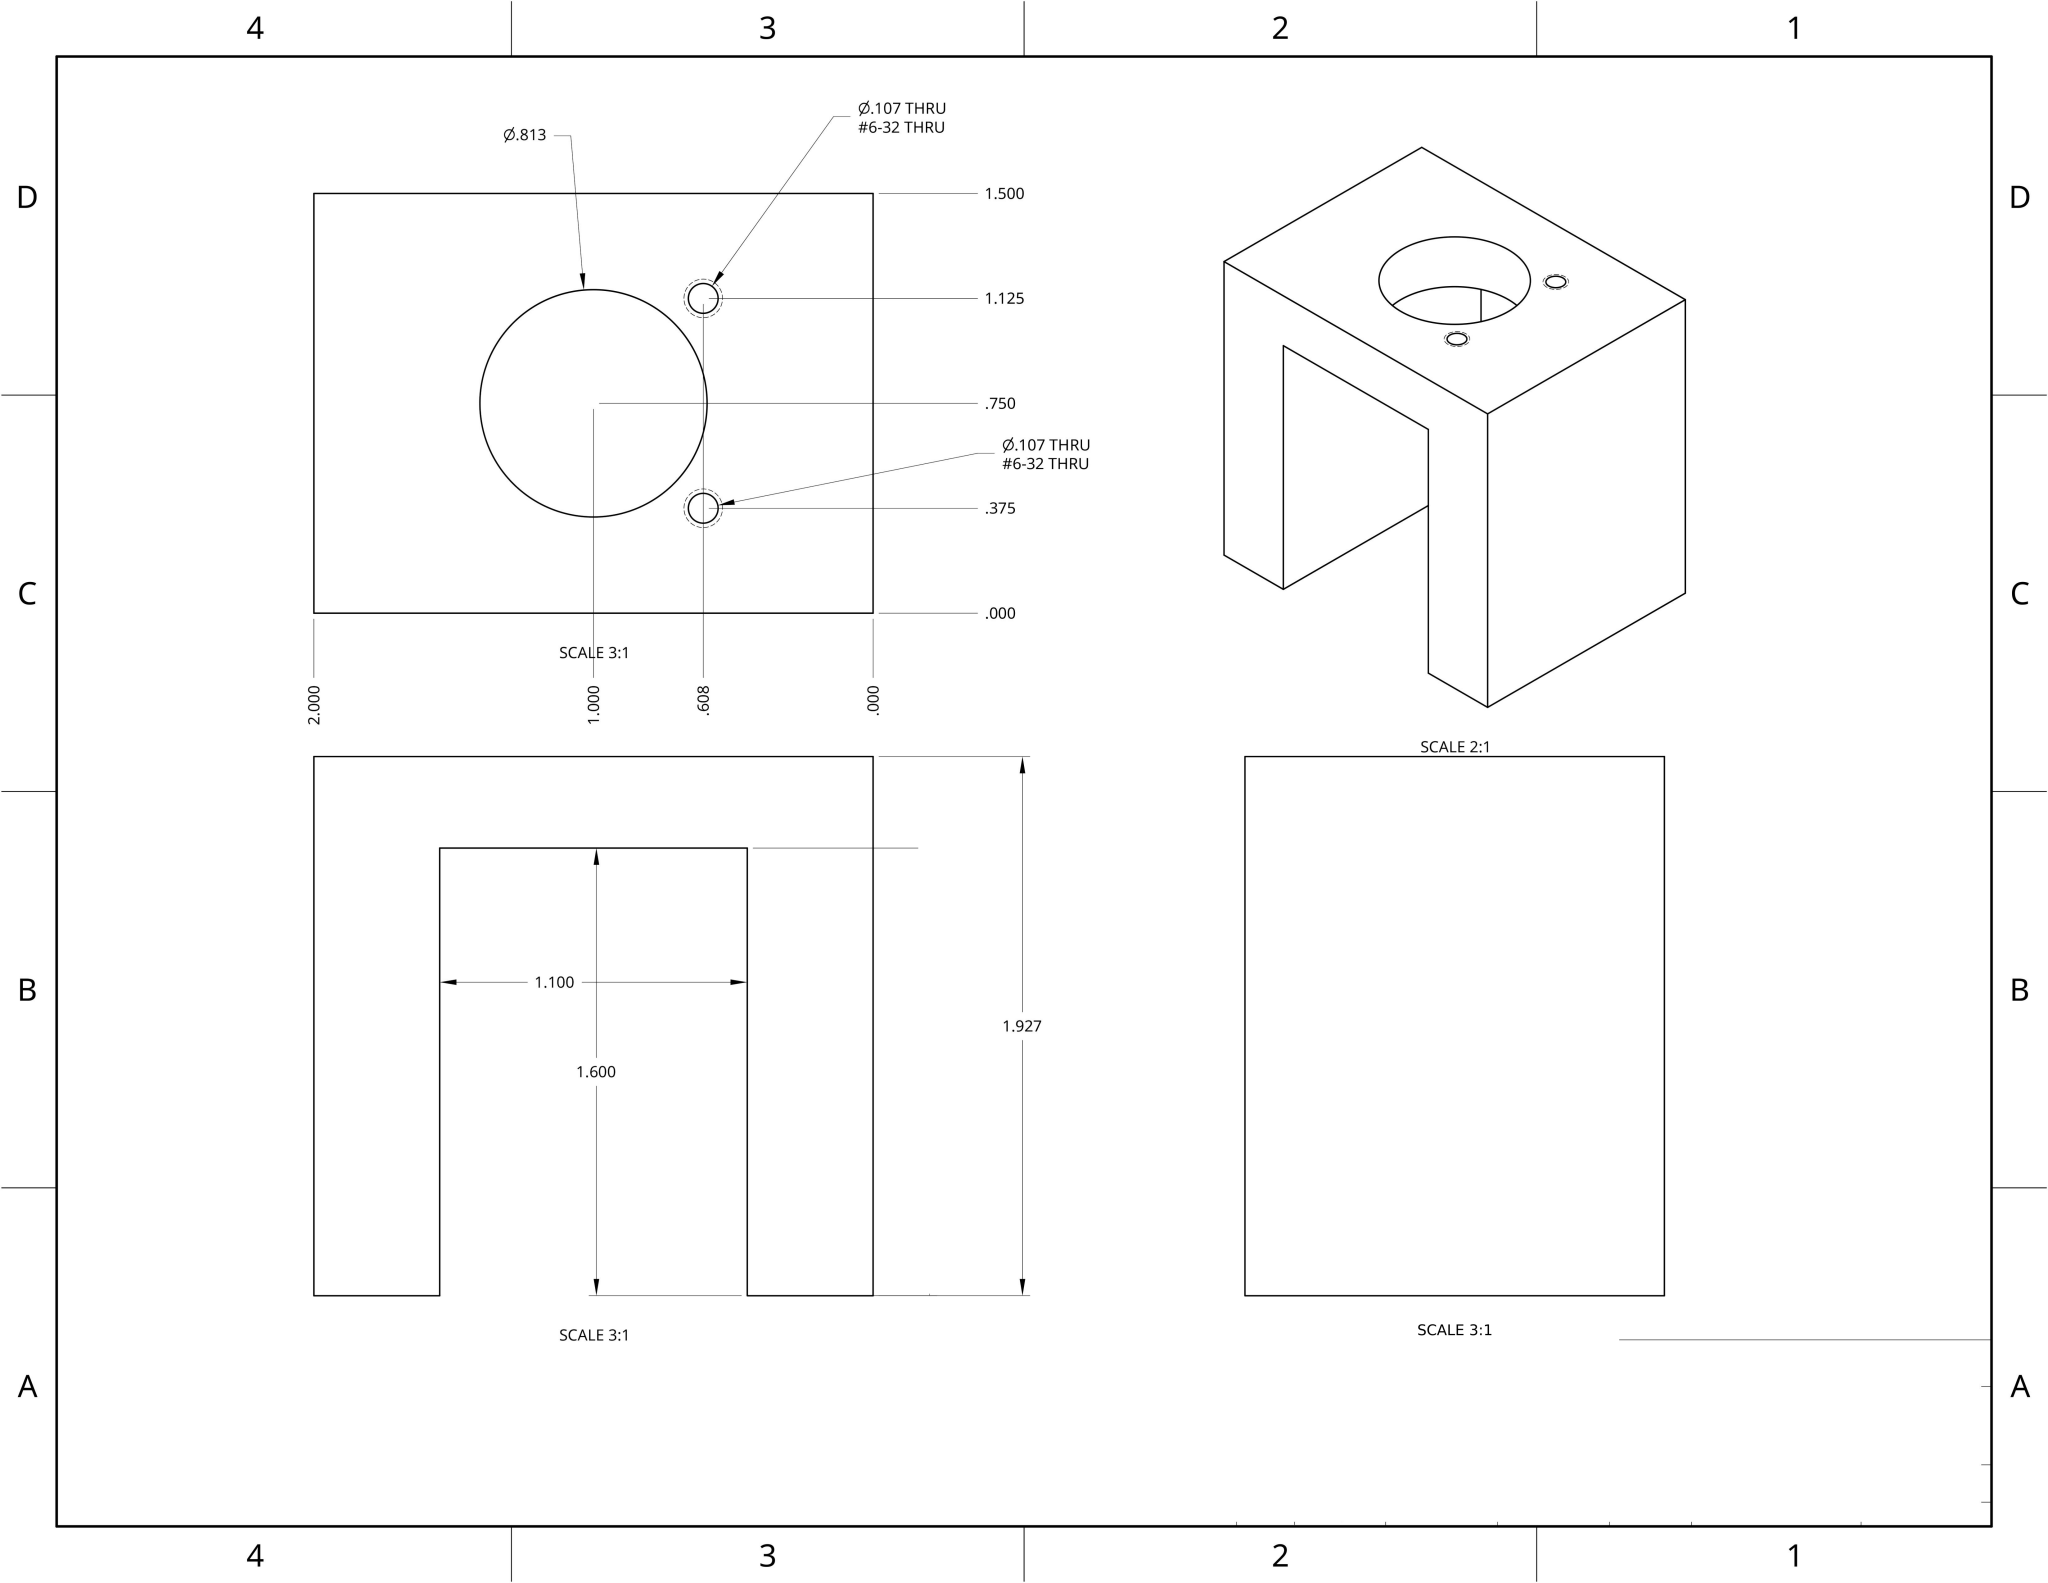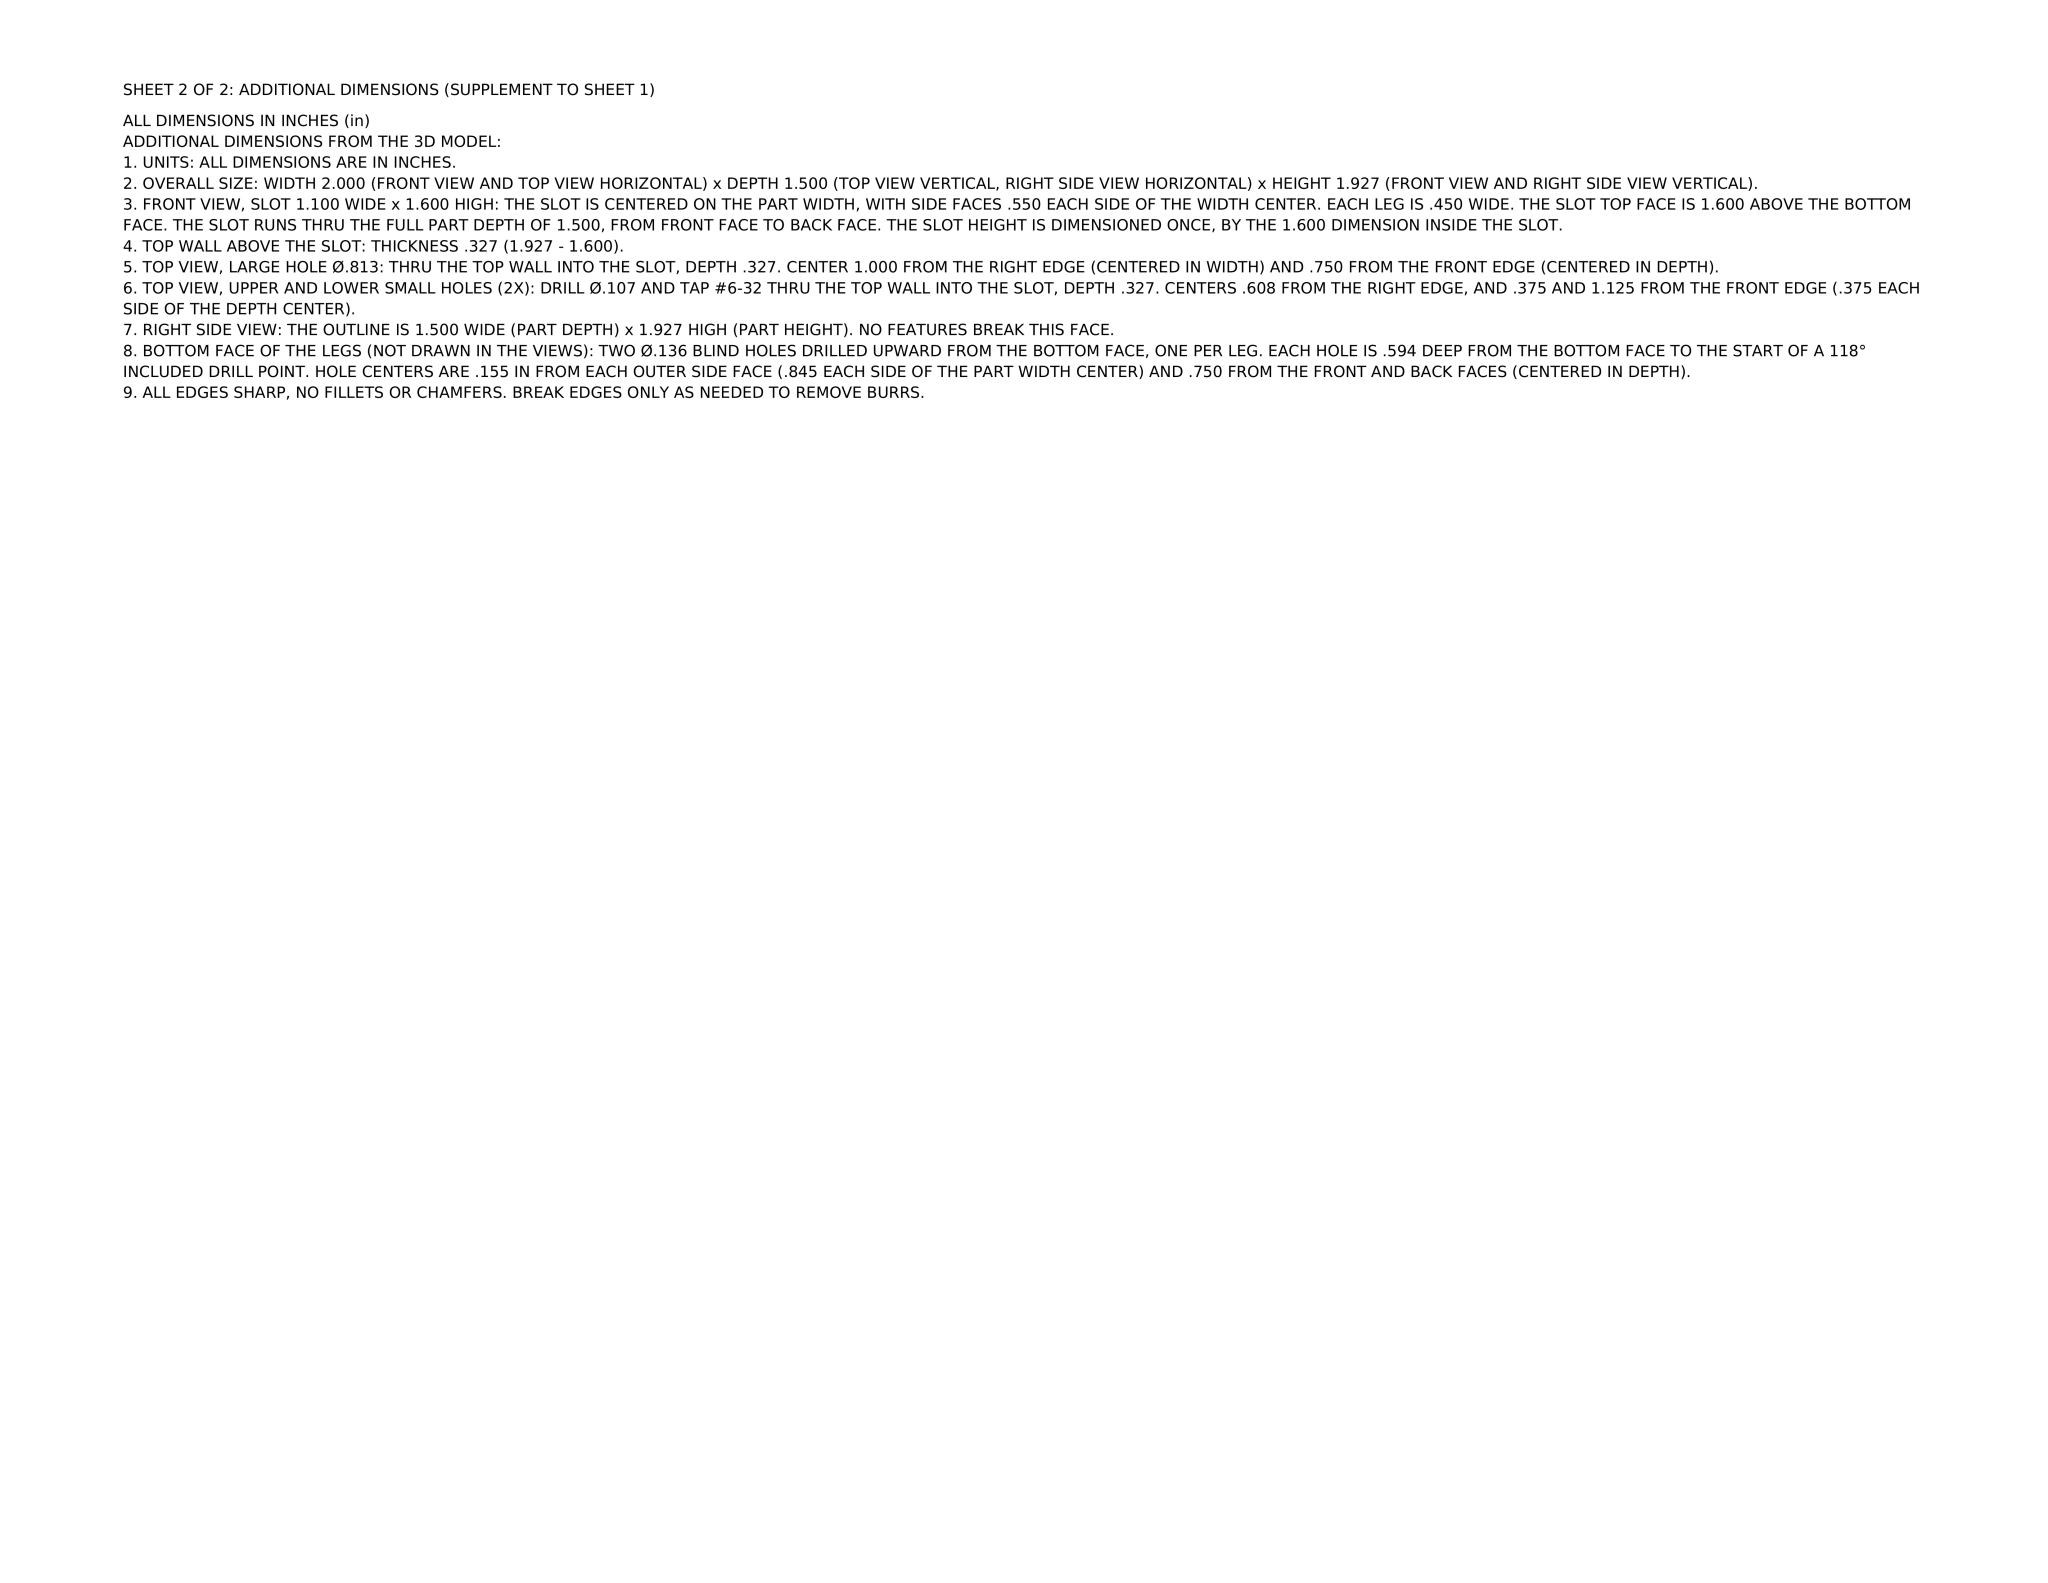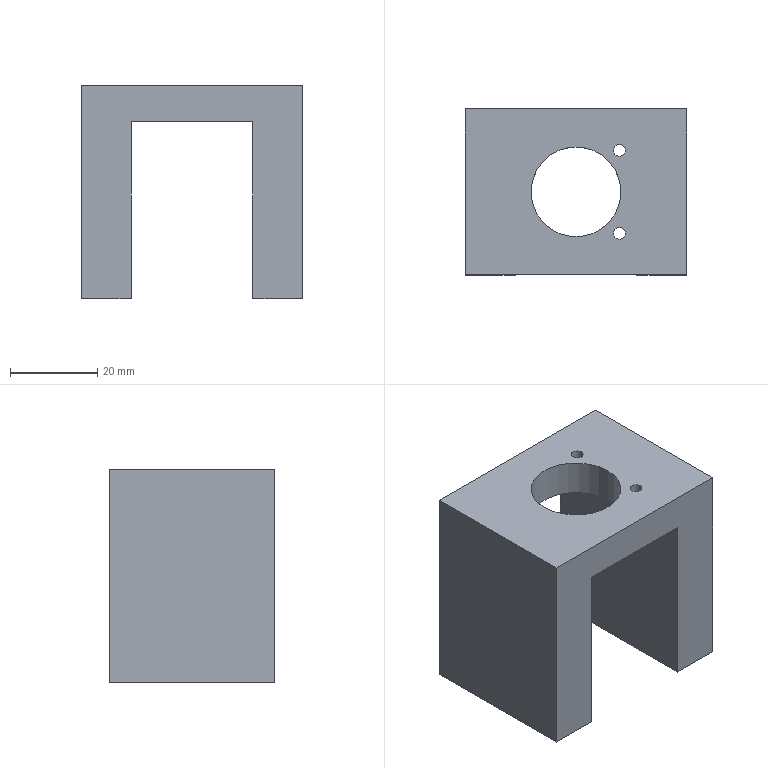Part | NX | drawing in metres | 1 solid | 17 faces | box 50.8 x 38.1 x 48.95 mm | volume 48309 mm3 | plane 10 | cylinder 5 | cone 2 | commonest cylinder face diameters 2.705 x2 3.454 x2 20.637 x1
STEP:
#1=COLOUR_RGB('',0.6039,0.6471,0.6863);
#2=FILL_AREA_STYLE_COLOUR('',#1);
#3=FILL_AREA_STYLE('',(#2));
#4=SURFACE_STYLE_FILL_AREA(#3);
#5=SURFACE_SIDE_STYLE('',(#4));
#6=SURFACE_STYLE_USAGE(.BOTH.,#5);
#7=PRESENTATION_STYLE_ASSIGNMENT((#6));
#8=CARTESIAN_POINT('',(0.01132,-0.009525,0.04895));
#9=VERTEX_POINT('',#8);
#10=CARTESIAN_POINT('',(0.009969,-0.009525,0.04895));
#11=DIRECTION('',(0.,0.,1.));
#12=DIRECTION('',(1.,0.,0.));
#13=AXIS2_PLACEMENT_3D('',#10,#11,#12);
#14=CIRCLE('',#13,0.001353);
#15=EDGE_CURVE('',#9,#9,#14,.F.);
#16=ORIENTED_EDGE('',*,*,#15,.F.);
#17=EDGE_LOOP('',(#16));
#18=FACE_OUTER_BOUND('',#17,.T.);
#19=CARTESIAN_POINT('',(0.01132,-0.009525,0.04064));
#20=VERTEX_POINT('',#19);
#21=CARTESIAN_POINT('',(0.009969,-0.009525,0.04064));
#22=DIRECTION('',(0.,0.,1.));
#23=DIRECTION('',(1.,0.,-0.));
#24=AXIS2_PLACEMENT_3D('',#21,#22,#23);
#25=CIRCLE('',#24,0.001353);
#26=EDGE_CURVE('',#20,#20,#25,.F.);
#27=ORIENTED_EDGE('',*,*,#26,.T.);
#28=EDGE_LOOP('',(#27));
#29=FACE_OUTER_BOUND('',#28,.T.);
#30=CARTESIAN_POINT('',(0.009969,-0.009525,0.08058));
#31=DIRECTION('',(0.,0.,1.));
#32=DIRECTION('',(-1.,0.,0.));
#33=AXIS2_PLACEMENT_3D('',#30,#31,#32);
#34=CYLINDRICAL_SURFACE('',#33,0.001353);
#35=ADVANCED_FACE('',(#18,#29),#34,.F.);
#36=STYLED_ITEM('',(#7),#35);
#37=COLOUR_RGB('',0.6039,0.6471,0.6863);
#38=FILL_AREA_STYLE_COLOUR('',#37);
#39=FILL_AREA_STYLE('',(#38));
#40=SURFACE_STYLE_FILL_AREA(#39);
#41=SURFACE_SIDE_STYLE('',(#40));
#42=SURFACE_STYLE_USAGE(.BOTH.,#41);
#43=PRESENTATION_STYLE_ASSIGNMENT((#42));
#44=CARTESIAN_POINT('',(-0.0254,0.01905,0.));
#45=VERTEX_POINT('',#44);
#46=CARTESIAN_POINT('',(-0.0254,-0.01905,0.));
#47=VERTEX_POINT('',#46);
#48=CARTESIAN_POINT('',(-0.0254,-0.004293,0.));
#49=DIRECTION('',(0.,-1.,0.));
#50=VECTOR('',#49,1.);
#51=LINE('',#48,#50);
#52=EDGE_CURVE('',#45,#47,#51,.T.);
#53=ORIENTED_EDGE('',*,*,#52,.T.);
#54=CARTESIAN_POINT('',(-0.0254,-0.01905,0.04895));
#55=VERTEX_POINT('',#54);
#56=CARTESIAN_POINT('',(-0.0254,-0.01905,0.04895));
#57=DIRECTION('',(0.,0.,-1.));
#58=VECTOR('',#57,1.);
#59=LINE('',#56,#58);
#60=EDGE_CURVE('',#55,#47,#59,.T.);
#61=ORIENTED_EDGE('',*,*,#60,.F.);
#62=CARTESIAN_POINT('',(-0.0254,0.01905,0.04895));
#63=VERTEX_POINT('',#62);
#64=CARTESIAN_POINT('',(-0.0254,-0.004293,0.04895));
#65=DIRECTION('',(0.,-1.,0.));
#66=VECTOR('',#65,1.);
#67=LINE('',#64,#66);
#68=EDGE_CURVE('',#63,#55,#67,.T.);
#69=ORIENTED_EDGE('',*,*,#68,.F.);
#70=CARTESIAN_POINT('',(-0.0254,0.01905,0.04895));
#71=DIRECTION('',(0.,0.,-1.));
#72=VECTOR('',#71,1.);
#73=LINE('',#70,#72);
#74=EDGE_CURVE('',#63,#45,#73,.T.);
#75=ORIENTED_EDGE('',*,*,#74,.T.);
#76=EDGE_LOOP('',(#53,#61,#69,#75));
#77=FACE_OUTER_BOUND('',#76,.T.);
#78=CARTESIAN_POINT('',(-0.0254,-0.004293,0.04895));
#79=DIRECTION('',(1.,0.,0.));
#80=DIRECTION('',(0.,0.,-1.));
#81=AXIS2_PLACEMENT_3D('',#78,#79,#80);
#82=PLANE('',#81);
#83=ADVANCED_FACE('',(#77),#82,.F.);
#84=STYLED_ITEM('',(#43),#83);
#85=COLOUR_RGB('',0.6039,0.6471,0.6863);
#86=FILL_AREA_STYLE_COLOUR('',#85);
#87=FILL_AREA_STYLE('',(#86));
#88=SURFACE_STYLE_FILL_AREA(#87);
#89=SURFACE_SIDE_STYLE('',(#88));
#90=SURFACE_STYLE_USAGE(.BOTH.,#89);
#91=PRESENTATION_STYLE_ASSIGNMENT((#90));
#92=CARTESIAN_POINT('',(0.01974,-0.,0.));
#93=VERTEX_POINT('',#92);
#94=CARTESIAN_POINT('',(0.02146,-0.,0.));
#95=DIRECTION('',(0.,0.,-1.));
#96=DIRECTION('',(-1.,0.,0.));
#97=AXIS2_PLACEMENT_3D('',#94,#95,#96);
#98=CIRCLE('',#97,0.001727);
#99=EDGE_CURVE('',#93,#93,#98,.T.);
#100=ORIENTED_EDGE('',*,*,#99,.F.);
#101=EDGE_LOOP('',(#100));
#102=FACE_BOUND('',#101,.T.);
#103=CARTESIAN_POINT('',(0.01397,-0.01905,-0.));
#104=VERTEX_POINT('',#103);
#105=CARTESIAN_POINT('',(0.0254,-0.01905,0.));
#106=VERTEX_POINT('',#105);
#107=CARTESIAN_POINT('',(0.01958,-0.01905,0.));
#108=DIRECTION('',(1.,0.,0.));
#109=VECTOR('',#108,1.);
#110=LINE('',#107,#109);
#111=EDGE_CURVE('',#104,#106,#110,.T.);
#112=ORIENTED_EDGE('',*,*,#111,.F.);
#113=CARTESIAN_POINT('',(0.01397,0.01905,-0.));
#114=VERTEX_POINT('',#113);
#115=CARTESIAN_POINT('',(0.01397,-0.06113,-0.));
#116=DIRECTION('',(-0.,1.,0.));
#117=VECTOR('',#116,1.);
#118=LINE('',#115,#117);
#119=EDGE_CURVE('',#104,#114,#118,.T.);
#120=ORIENTED_EDGE('',*,*,#119,.T.);
#121=CARTESIAN_POINT('',(0.0254,0.01905,0.));
#122=VERTEX_POINT('',#121);
#123=CARTESIAN_POINT('',(0.01958,0.01905,0.));
#124=DIRECTION('',(1.,0.,0.));
#125=VECTOR('',#124,1.);
#126=LINE('',#123,#125);
#127=EDGE_CURVE('',#114,#122,#126,.T.);
#128=ORIENTED_EDGE('',*,*,#127,.T.);
#129=CARTESIAN_POINT('',(0.0254,-0.004293,0.));
#130=DIRECTION('',(0.,-1.,0.));
#131=VECTOR('',#130,1.);
#132=LINE('',#129,#131);
#133=EDGE_CURVE('',#122,#106,#132,.T.);
#134=ORIENTED_EDGE('',*,*,#133,.T.);
#135=EDGE_LOOP('',(#112,#120,#128,#134));
#136=FACE_OUTER_BOUND('',#135,.T.);
#137=CARTESIAN_POINT('',(0.,-0.,0.));
#138=DIRECTION('',(0.,0.,1.));
#139=DIRECTION('',(1.,0.,0.));
#140=AXIS2_PLACEMENT_3D('',#137,#138,#139);
#141=PLANE('',#140);
#142=ADVANCED_FACE('',(#102,#136),#141,.F.);
#143=STYLED_ITEM('',(#91),#142);
#144=COLOUR_RGB('',0.6039,0.6471,0.6863);
#145=FILL_AREA_STYLE_COLOUR('',#144);
#146=FILL_AREA_STYLE('',(#145));
#147=SURFACE_STYLE_FILL_AREA(#146);
#148=SURFACE_SIDE_STYLE('',(#147));
#149=SURFACE_STYLE_USAGE(.BOTH.,#148);
#150=PRESENTATION_STYLE_ASSIGNMENT((#149));
#151=CARTESIAN_POINT('',(0.01974,-0.,0.01508));
#152=VERTEX_POINT('',#151);
#153=CARTESIAN_POINT('',(0.02146,-0.,0.01508));
#154=DIRECTION('',(0.,0.,-1.));
#155=DIRECTION('',(-1.,0.,0.));
#156=AXIS2_PLACEMENT_3D('',#153,#154,#155);
#157=CIRCLE('',#156,0.001727);
#158=EDGE_CURVE('',#152,#152,#157,.T.);
#159=ORIENTED_EDGE('',*,*,#158,.T.);
#160=EDGE_LOOP('',(#159));
#161=FACE_OUTER_BOUND('',#160,.T.);
#162=CARTESIAN_POINT('',(0.02146,-0.,0.01612));
#163=VERTEX_POINT('',#162);
#164=VERTEX_LOOP('',#163);
#165=FACE_BOUND('',#164,.T.);
#166=CARTESIAN_POINT('',(0.02146,-0.,-0.4989));
#167=DIRECTION('',(0.,0.,-1.));
#168=DIRECTION('',(-1.,0.,0.));
#169=AXIS2_PLACEMENT_3D('',#166,#167,#168);
#170=CONICAL_SURFACE('',#169,0.8572,1.03);
#171=ADVANCED_FACE('',(#161,#165),#170,.F.);
#172=STYLED_ITEM('',(#150),#171);
#173=COLOUR_RGB('',0.6039,0.6471,0.6863);
#174=FILL_AREA_STYLE_COLOUR('',#173);
#175=FILL_AREA_STYLE('',(#174));
#176=SURFACE_STYLE_FILL_AREA(#175);
#177=SURFACE_SIDE_STYLE('',(#176));
#178=SURFACE_STYLE_USAGE(.BOTH.,#177);
#179=PRESENTATION_STYLE_ASSIGNMENT((#178));
#180=ORIENTED_EDGE('',*,*,#26,.F.);
#181=EDGE_LOOP('',(#180));
#182=FACE_BOUND('',#181,.T.);
#183=CARTESIAN_POINT('',(0.01132,0.009525,0.04064));
#184=VERTEX_POINT('',#183);
#185=CARTESIAN_POINT('',(0.009969,0.009525,0.04064));
#186=DIRECTION('',(0.,0.,1.));
#187=DIRECTION('',(1.,0.,-0.));
#188=AXIS2_PLACEMENT_3D('',#185,#186,#187);
#189=CIRCLE('',#188,0.001353);
#190=EDGE_CURVE('',#184,#184,#189,.F.);
#191=ORIENTED_EDGE('',*,*,#190,.F.);
#192=EDGE_LOOP('',(#191));
#193=FACE_BOUND('',#192,.T.);
#194=CARTESIAN_POINT('',(0.01032,0.,0.04064));
#195=VERTEX_POINT('',#194);
#196=CARTESIAN_POINT('',(0.,0.,0.04064));
#197=DIRECTION('',(0.,0.,1.));
#198=DIRECTION('',(1.,0.,-0.));
#199=AXIS2_PLACEMENT_3D('',#196,#197,#198);
#200=CIRCLE('',#199,0.01032);
#201=EDGE_CURVE('',#195,#195,#200,.T.);
#202=ORIENTED_EDGE('',*,*,#201,.T.);
#203=EDGE_LOOP('',(#202));
#204=FACE_BOUND('',#203,.T.);
#205=CARTESIAN_POINT('',(-0.01397,-0.01905,0.04064));
#206=VERTEX_POINT('',#205);
#207=CARTESIAN_POINT('',(-0.01397,0.01905,0.04064));
#208=VERTEX_POINT('',#207);
#209=CARTESIAN_POINT('',(-0.01397,-0.06113,0.04064));
#210=DIRECTION('',(-0.,1.,0.));
#211=VECTOR('',#210,1.);
#212=LINE('',#209,#211);
#213=EDGE_CURVE('',#206,#208,#212,.T.);
#214=ORIENTED_EDGE('',*,*,#213,.T.);
#215=CARTESIAN_POINT('',(0.01397,0.01905,0.04064));
#216=VERTEX_POINT('',#215);
#217=CARTESIAN_POINT('',(-0.02417,0.01905,0.04064));
#218=DIRECTION('',(1.,0.,-0.));
#219=VECTOR('',#218,1.);
#220=LINE('',#217,#219);
#221=EDGE_CURVE('',#208,#216,#220,.T.);
#222=ORIENTED_EDGE('',*,*,#221,.T.);
#223=CARTESIAN_POINT('',(0.01397,-0.01905,0.04064));
#224=VERTEX_POINT('',#223);
#225=CARTESIAN_POINT('',(0.01397,-0.06113,0.04064));
#226=DIRECTION('',(-0.,1.,0.));
#227=VECTOR('',#226,1.);
#228=LINE('',#225,#227);
#229=EDGE_CURVE('',#224,#216,#228,.T.);
#230=ORIENTED_EDGE('',*,*,#229,.F.);
#231=CARTESIAN_POINT('',(0.01958,-0.01905,0.04064));
#232=DIRECTION('',(1.,0.,-0.));
#233=VECTOR('',#232,1.);
#234=LINE('',#231,#233);
#235=EDGE_CURVE('',#206,#224,#234,.T.);
#236=ORIENTED_EDGE('',*,*,#235,.F.);
#237=EDGE_LOOP('',(#214,#222,#230,#236));
#238=FACE_OUTER_BOUND('',#237,.T.);
#239=CARTESIAN_POINT('',(-0.02417,-0.06113,0.04064));
#240=DIRECTION('',(0.,0.,1.));
#241=DIRECTION('',(1.,0.,-0.));
#242=AXIS2_PLACEMENT_3D('',#239,#240,#241);
#243=PLANE('',#242);
#244=ADVANCED_FACE('',(#182,#193,#204,#238),#243,.F.);
#245=STYLED_ITEM('',(#179),#244);
#246=COLOUR_RGB('',0.6039,0.6471,0.6863);
#247=FILL_AREA_STYLE_COLOUR('',#246);
#248=FILL_AREA_STYLE('',(#247));
#249=SURFACE_STYLE_FILL_AREA(#248);
#250=SURFACE_SIDE_STYLE('',(#249));
#251=SURFACE_STYLE_USAGE(.BOTH.,#250);
#252=PRESENTATION_STYLE_ASSIGNMENT((#251));
#253=CARTESIAN_POINT('',(-0.01397,-0.01905,-0.));
#254=VERTEX_POINT('',#253);
#255=CARTESIAN_POINT('',(-0.01397,0.01905,-0.));
#256=VERTEX_POINT('',#255);
#257=CARTESIAN_POINT('',(-0.01397,-0.06113,-0.));
#258=DIRECTION('',(-0.,1.,0.));
#259=VECTOR('',#258,1.);
#260=LINE('',#257,#259);
#261=EDGE_CURVE('',#254,#256,#260,.T.);
#262=ORIENTED_EDGE('',*,*,#261,.T.);
#263=CARTESIAN_POINT('',(-0.01397,0.01905,0.004866));
#264=DIRECTION('',(0.,0.,1.));
#265=VECTOR('',#264,1.);
#266=LINE('',#263,#265);
#267=EDGE_CURVE('',#256,#208,#266,.T.);
#268=ORIENTED_EDGE('',*,*,#267,.T.);
#269=ORIENTED_EDGE('',*,*,#213,.F.);
#270=CARTESIAN_POINT('',(-0.01397,-0.01905,0.04895));
#271=DIRECTION('',(0.,0.,1.));
#272=VECTOR('',#271,1.);
#273=LINE('',#270,#272);
#274=EDGE_CURVE('',#254,#206,#273,.T.);
#275=ORIENTED_EDGE('',*,*,#274,.F.);
#276=EDGE_LOOP('',(#262,#268,#269,#275));
#277=FACE_OUTER_BOUND('',#276,.T.);
#278=CARTESIAN_POINT('',(-0.01397,-0.06113,0.004866));
#279=DIRECTION('',(-1.,-0.,0.));
#280=DIRECTION('',(0.,0.,1.));
#281=AXIS2_PLACEMENT_3D('',#278,#279,#280);
#282=PLANE('',#281);
#283=ADVANCED_FACE('',(#277),#282,.F.);
#284=STYLED_ITEM('',(#252),#283);
#285=COLOUR_RGB('',0.6039,0.6471,0.6863);
#286=FILL_AREA_STYLE_COLOUR('',#285);
#287=FILL_AREA_STYLE('',(#286));
#288=SURFACE_STYLE_FILL_AREA(#287);
#289=SURFACE_SIDE_STYLE('',(#288));
#290=SURFACE_STYLE_USAGE(.BOTH.,#289);
#291=PRESENTATION_STYLE_ASSIGNMENT((#290));
#292=ORIENTED_EDGE('',*,*,#15,.T.);
#293=EDGE_LOOP('',(#292));
#294=FACE_BOUND('',#293,.T.);
#295=CARTESIAN_POINT('',(0.01132,0.009525,0.04895));
#296=VERTEX_POINT('',#295);
#297=CARTESIAN_POINT('',(0.009969,0.009525,0.04895));
#298=DIRECTION('',(0.,0.,1.));
#299=DIRECTION('',(1.,0.,0.));
#300=AXIS2_PLACEMENT_3D('',#297,#298,#299);
#301=CIRCLE('',#300,0.001353);
#302=EDGE_CURVE('',#296,#296,#301,.F.);
#303=ORIENTED_EDGE('',*,*,#302,.T.);
#304=EDGE_LOOP('',(#303));
#305=FACE_BOUND('',#304,.T.);
#306=CARTESIAN_POINT('',(0.01032,0.,0.04895));
#307=VERTEX_POINT('',#306);
#308=CARTESIAN_POINT('',(0.,0.,0.04895));
#309=DIRECTION('',(0.,0.,1.));
#310=DIRECTION('',(1.,0.,0.));
#311=AXIS2_PLACEMENT_3D('',#308,#309,#310);
#312=CIRCLE('',#311,0.01032);
#313=EDGE_CURVE('',#307,#307,#312,.T.);
#314=ORIENTED_EDGE('',*,*,#313,.F.);
#315=EDGE_LOOP('',(#314));
#316=FACE_BOUND('',#315,.T.);
#317=ORIENTED_EDGE('',*,*,#68,.T.);
#318=CARTESIAN_POINT('',(0.0254,-0.01905,0.04895));
#319=VERTEX_POINT('',#318);
#320=CARTESIAN_POINT('',(0.01958,-0.01905,0.04895));
#321=DIRECTION('',(1.,0.,0.));
#322=VECTOR('',#321,1.);
#323=LINE('',#320,#322);
#324=EDGE_CURVE('',#55,#319,#323,.T.);
#325=ORIENTED_EDGE('',*,*,#324,.T.);
#326=CARTESIAN_POINT('',(0.0254,0.01905,0.04895));
#327=VERTEX_POINT('',#326);
#328=CARTESIAN_POINT('',(0.0254,-0.004293,0.04895));
#329=DIRECTION('',(0.,-1.,0.));
#330=VECTOR('',#329,1.);
#331=LINE('',#328,#330);
#332=EDGE_CURVE('',#327,#319,#331,.T.);
#333=ORIENTED_EDGE('',*,*,#332,.F.);
#334=CARTESIAN_POINT('',(0.01958,0.01905,0.04895));
#335=DIRECTION('',(1.,0.,0.));
#336=VECTOR('',#335,1.);
#337=LINE('',#334,#336);
#338=EDGE_CURVE('',#63,#327,#337,.T.);
#339=ORIENTED_EDGE('',*,*,#338,.F.);
#340=EDGE_LOOP('',(#317,#325,#333,#339));
#341=FACE_OUTER_BOUND('',#340,.T.);
#342=CARTESIAN_POINT('',(0.,-0.,0.04895));
#343=DIRECTION('',(0.,0.,1.));
#344=DIRECTION('',(1.,0.,0.));
#345=AXIS2_PLACEMENT_3D('',#342,#343,#344);
#346=PLANE('',#345);
#347=ADVANCED_FACE('',(#294,#305,#316,#341),#346,.T.);
#348=STYLED_ITEM('',(#291),#347);
#349=COLOUR_RGB('',0.6039,0.6471,0.6863);
#350=FILL_AREA_STYLE_COLOUR('',#349);
#351=FILL_AREA_STYLE('',(#350));
#352=SURFACE_STYLE_FILL_AREA(#351);
#353=SURFACE_SIDE_STYLE('',(#352));
#354=SURFACE_STYLE_USAGE(.BOTH.,#353);
#355=PRESENTATION_STYLE_ASSIGNMENT((#354));
#356=CARTESIAN_POINT('',(-0.02319,0.,0.));
#357=VERTEX_POINT('',#356);
#358=CARTESIAN_POINT('',(-0.02146,0.,0.));
#359=DIRECTION('',(0.,0.,-1.));
#360=DIRECTION('',(-1.,0.,0.));
#361=AXIS2_PLACEMENT_3D('',#358,#359,#360);
#362=CIRCLE('',#361,0.001727);
#363=EDGE_CURVE('',#357,#357,#362,.T.);
#364=ORIENTED_EDGE('',*,*,#363,.F.);
#365=EDGE_LOOP('',(#364));
#366=FACE_BOUND('',#365,.T.);
#367=ORIENTED_EDGE('',*,*,#261,.F.);
#368=CARTESIAN_POINT('',(0.01958,-0.01905,0.));
#369=DIRECTION('',(1.,0.,0.));
#370=VECTOR('',#369,1.);
#371=LINE('',#368,#370);
#372=EDGE_CURVE('',#47,#254,#371,.T.);
#373=ORIENTED_EDGE('',*,*,#372,.F.);
#374=ORIENTED_EDGE('',*,*,#52,.F.);
#375=CARTESIAN_POINT('',(0.01958,0.01905,0.));
#376=DIRECTION('',(1.,0.,0.));
#377=VECTOR('',#376,1.);
#378=LINE('',#375,#377);
#379=EDGE_CURVE('',#45,#256,#378,.T.);
#380=ORIENTED_EDGE('',*,*,#379,.T.);
#381=EDGE_LOOP('',(#367,#373,#374,#380));
#382=FACE_OUTER_BOUND('',#381,.T.);
#383=CARTESIAN_POINT('',(0.,-0.,0.));
#384=DIRECTION('',(0.,0.,1.));
#385=DIRECTION('',(1.,0.,0.));
#386=AXIS2_PLACEMENT_3D('',#383,#384,#385);
#387=PLANE('',#386);
#388=ADVANCED_FACE('',(#366,#382),#387,.F.);
#389=STYLED_ITEM('',(#355),#388);
#390=COLOUR_RGB('',0.6039,0.6471,0.6863);
#391=FILL_AREA_STYLE_COLOUR('',#390);
#392=FILL_AREA_STYLE('',(#391));
#393=SURFACE_STYLE_FILL_AREA(#392);
#394=SURFACE_SIDE_STYLE('',(#393));
#395=SURFACE_STYLE_USAGE(.BOTH.,#394);
#396=PRESENTATION_STYLE_ASSIGNMENT((#395));
#397=ORIENTED_EDGE('',*,*,#99,.T.);
#398=EDGE_LOOP('',(#397));
#399=FACE_OUTER_BOUND('',#398,.T.);
#400=ORIENTED_EDGE('',*,*,#158,.F.);
#401=EDGE_LOOP('',(#400));
#402=FACE_OUTER_BOUND('',#401,.T.);
#403=CARTESIAN_POINT('',(0.02146,-0.,0.00806));
#404=DIRECTION('',(0.,0.,1.));
#405=DIRECTION('',(-1.,0.,0.));
#406=AXIS2_PLACEMENT_3D('',#403,#404,#405);
#407=CYLINDRICAL_SURFACE('',#406,0.001727);
#408=ADVANCED_FACE('',(#399,#402),#407,.F.);
#409=STYLED_ITEM('',(#396),#408);
#410=COLOUR_RGB('',0.6039,0.6471,0.6863);
#411=FILL_AREA_STYLE_COLOUR('',#410);
#412=FILL_AREA_STYLE('',(#411));
#413=SURFACE_STYLE_FILL_AREA(#412);
#414=SURFACE_SIDE_STYLE('',(#413));
#415=SURFACE_STYLE_USAGE(.BOTH.,#414);
#416=PRESENTATION_STYLE_ASSIGNMENT((#415));
#417=ORIENTED_EDGE('',*,*,#302,.F.);
#418=EDGE_LOOP('',(#417));
#419=FACE_OUTER_BOUND('',#418,.T.);
#420=ORIENTED_EDGE('',*,*,#190,.T.);
#421=EDGE_LOOP('',(#420));
#422=FACE_OUTER_BOUND('',#421,.T.);
#423=CARTESIAN_POINT('',(0.009969,0.009525,0.08058));
#424=DIRECTION('',(0.,0.,1.));
#425=DIRECTION('',(-1.,0.,0.));
#426=AXIS2_PLACEMENT_3D('',#423,#424,#425);
#427=CYLINDRICAL_SURFACE('',#426,0.001353);
#428=ADVANCED_FACE('',(#419,#422),#427,.F.);
#429=STYLED_ITEM('',(#416),#428);
#430=COLOUR_RGB('',0.6039,0.6471,0.6863);
#431=FILL_AREA_STYLE_COLOUR('',#430);
#432=FILL_AREA_STYLE('',(#431));
#433=SURFACE_STYLE_FILL_AREA(#432);
#434=SURFACE_SIDE_STYLE('',(#433));
#435=SURFACE_STYLE_USAGE(.BOTH.,#434);
#436=PRESENTATION_STYLE_ASSIGNMENT((#435));
#437=CARTESIAN_POINT('',(0.01397,-0.01905,0.04895));
#438=DIRECTION('',(0.,0.,1.));
#439=VECTOR('',#438,1.);
#440=LINE('',#437,#439);
#441=EDGE_CURVE('',#104,#224,#440,.T.);
#442=ORIENTED_EDGE('',*,*,#441,.T.);
#443=ORIENTED_EDGE('',*,*,#229,.T.);
#444=CARTESIAN_POINT('',(0.01397,0.01905,0.004866));
#445=DIRECTION('',(0.,0.,1.));
#446=VECTOR('',#445,1.);
#447=LINE('',#444,#446);
#448=EDGE_CURVE('',#114,#216,#447,.T.);
#449=ORIENTED_EDGE('',*,*,#448,.F.);
#450=ORIENTED_EDGE('',*,*,#119,.F.);
#451=EDGE_LOOP('',(#442,#443,#449,#450));
#452=FACE_OUTER_BOUND('',#451,.T.);
#453=CARTESIAN_POINT('',(0.01397,-0.06113,0.004866));
#454=DIRECTION('',(-1.,-0.,0.));
#455=DIRECTION('',(0.,0.,1.));
#456=AXIS2_PLACEMENT_3D('',#453,#454,#455);
#457=PLANE('',#456);
#458=ADVANCED_FACE('',(#452),#457,.T.);
#459=STYLED_ITEM('',(#436),#458);
#460=COLOUR_RGB('',0.6039,0.6471,0.6863);
#461=FILL_AREA_STYLE_COLOUR('',#460);
#462=FILL_AREA_STYLE('',(#461));
#463=SURFACE_STYLE_FILL_AREA(#462);
#464=SURFACE_SIDE_STYLE('',(#463));
#465=SURFACE_STYLE_USAGE(.BOTH.,#464);
#466=PRESENTATION_STYLE_ASSIGNMENT((#465));
#467=ORIENTED_EDGE('',*,*,#363,.T.);
#468=EDGE_LOOP('',(#467));
#469=FACE_OUTER_BOUND('',#468,.T.);
#470=CARTESIAN_POINT('',(-0.02319,0.,0.01508));
#471=VERTEX_POINT('',#470);
#472=CARTESIAN_POINT('',(-0.02146,0.,0.01508));
#473=DIRECTION('',(0.,0.,-1.));
#474=DIRECTION('',(-1.,0.,0.));
#475=AXIS2_PLACEMENT_3D('',#472,#473,#474);
#476=CIRCLE('',#475,0.001727);
#477=EDGE_CURVE('',#471,#471,#476,.T.);
#478=ORIENTED_EDGE('',*,*,#477,.F.);
#479=EDGE_LOOP('',(#478));
#480=FACE_OUTER_BOUND('',#479,.T.);
#481=CARTESIAN_POINT('',(-0.02146,0.,0.00806));
#482=DIRECTION('',(0.,0.,1.));
#483=DIRECTION('',(-1.,0.,0.));
#484=AXIS2_PLACEMENT_3D('',#481,#482,#483);
#485=CYLINDRICAL_SURFACE('',#484,0.001727);
#486=ADVANCED_FACE('',(#469,#480),#485,.F.);
#487=STYLED_ITEM('',(#466),#486);
#488=COLOUR_RGB('',0.6039,0.6471,0.6863);
#489=FILL_AREA_STYLE_COLOUR('',#488);
#490=FILL_AREA_STYLE('',(#489));
#491=SURFACE_STYLE_FILL_AREA(#490);
#492=SURFACE_SIDE_STYLE('',(#491));
#493=SURFACE_STYLE_USAGE(.BOTH.,#492);
#494=PRESENTATION_STYLE_ASSIGNMENT((#493));
#495=ORIENTED_EDGE('',*,*,#267,.F.);
#496=ORIENTED_EDGE('',*,*,#379,.F.);
#497=ORIENTED_EDGE('',*,*,#74,.F.);
#498=ORIENTED_EDGE('',*,*,#338,.T.);
#499=CARTESIAN_POINT('',(0.0254,0.01905,0.04895));
#500=DIRECTION('',(0.,0.,-1.));
#501=VECTOR('',#500,1.);
#502=LINE('',#499,#501);
#503=EDGE_CURVE('',#327,#122,#502,.T.);
#504=ORIENTED_EDGE('',*,*,#503,.T.);
#505=ORIENTED_EDGE('',*,*,#127,.F.);
#506=ORIENTED_EDGE('',*,*,#448,.T.);
#507=ORIENTED_EDGE('',*,*,#221,.F.);
#508=EDGE_LOOP('',(#495,#496,#497,#498,#504,#505,#506,#507));
#509=FACE_OUTER_BOUND('',#508,.T.);
#510=CARTESIAN_POINT('',(0.01958,0.01905,0.04895));
#511=DIRECTION('',(-0.,1.,0.));
#512=DIRECTION('',(-1.,-0.,0.));
#513=AXIS2_PLACEMENT_3D('',#510,#511,#512);
#514=PLANE('',#513);
#515=ADVANCED_FACE('',(#509),#514,.T.);
#516=STYLED_ITEM('',(#494),#515);
#517=COLOUR_RGB('',0.6039,0.6471,0.6863);
#518=FILL_AREA_STYLE_COLOUR('',#517);
#519=FILL_AREA_STYLE('',(#518));
#520=SURFACE_STYLE_FILL_AREA(#519);
#521=SURFACE_SIDE_STYLE('',(#520));
#522=SURFACE_STYLE_USAGE(.BOTH.,#521);
#523=PRESENTATION_STYLE_ASSIGNMENT((#522));
#524=ORIENTED_EDGE('',*,*,#372,.T.);
#525=ORIENTED_EDGE('',*,*,#274,.T.);
#526=ORIENTED_EDGE('',*,*,#235,.T.);
#527=ORIENTED_EDGE('',*,*,#441,.F.);
#528=ORIENTED_EDGE('',*,*,#111,.T.);
#529=CARTESIAN_POINT('',(0.0254,-0.01905,0.04895));
#530=DIRECTION('',(0.,0.,-1.));
#531=VECTOR('',#530,1.);
#532=LINE('',#529,#531);
#533=EDGE_CURVE('',#319,#106,#532,.T.);
#534=ORIENTED_EDGE('',*,*,#533,.F.);
#535=ORIENTED_EDGE('',*,*,#324,.F.);
#536=ORIENTED_EDGE('',*,*,#60,.T.);
#537=EDGE_LOOP('',(#524,#525,#526,#527,#528,#534,#535,#536));
#538=FACE_OUTER_BOUND('',#537,.T.);
#539=CARTESIAN_POINT('',(0.01958,-0.01905,0.04895));
#540=DIRECTION('',(-0.,1.,0.));
#541=DIRECTION('',(-1.,-0.,0.));
#542=AXIS2_PLACEMENT_3D('',#539,#540,#541);
#543=PLANE('',#542);
#544=ADVANCED_FACE('',(#538),#543,.F.);
#545=STYLED_ITEM('',(#523),#544);
#546=COLOUR_RGB('',0.6039,0.6471,0.6863);
#547=FILL_AREA_STYLE_COLOUR('',#546);
#548=FILL_AREA_STYLE('',(#547));
#549=SURFACE_STYLE_FILL_AREA(#548);
#550=SURFACE_SIDE_STYLE('',(#549));
#551=SURFACE_STYLE_USAGE(.BOTH.,#550);
#552=PRESENTATION_STYLE_ASSIGNMENT((#551));
#553=ORIENTED_EDGE('',*,*,#477,.T.);
#554=EDGE_LOOP('',(#553));
#555=FACE_OUTER_BOUND('',#554,.T.);
#556=CARTESIAN_POINT('',(-0.02146,0.,0.01612));
#557=VERTEX_POINT('',#556);
#558=VERTEX_LOOP('',#557);
#559=FACE_BOUND('',#558,.T.);
#560=CARTESIAN_POINT('',(-0.02146,0.,-0.4989));
#561=DIRECTION('',(0.,0.,-1.));
#562=DIRECTION('',(-1.,0.,0.));
#563=AXIS2_PLACEMENT_3D('',#560,#561,#562);
#564=CONICAL_SURFACE('',#563,0.8572,1.03);
#565=ADVANCED_FACE('',(#555,#559),#564,.F.);
#566=STYLED_ITEM('',(#552),#565);
#567=COLOUR_RGB('',0.6039,0.6471,0.6863);
#568=FILL_AREA_STYLE_COLOUR('',#567);
#569=FILL_AREA_STYLE('',(#568));
#570=SURFACE_STYLE_FILL_AREA(#569);
#571=SURFACE_SIDE_STYLE('',(#570));
#572=SURFACE_STYLE_USAGE(.BOTH.,#571);
#573=PRESENTATION_STYLE_ASSIGNMENT((#572));
#574=ORIENTED_EDGE('',*,*,#201,.F.);
#575=EDGE_LOOP('',(#574));
#576=FACE_OUTER_BOUND('',#575,.T.);
#577=ORIENTED_EDGE('',*,*,#313,.T.);
#578=EDGE_LOOP('',(#577));
#579=FACE_OUTER_BOUND('',#578,.T.);
#580=CARTESIAN_POINT('',(0.,0.,0.04895));
#581=DIRECTION('',(0.,0.,1.));
#582=DIRECTION('',(-1.,0.,0.));
#583=AXIS2_PLACEMENT_3D('',#580,#581,#582);
#584=CYLINDRICAL_SURFACE('',#583,0.01032);
#585=ADVANCED_FACE('',(#576,#579),#584,.F.);
#586=STYLED_ITEM('',(#573),#585);
#587=COLOUR_RGB('',0.6039,0.6471,0.6863);
#588=FILL_AREA_STYLE_COLOUR('',#587);
#589=FILL_AREA_STYLE('',(#588));
#590=SURFACE_STYLE_FILL_AREA(#589);
#591=SURFACE_SIDE_STYLE('',(#590));
#592=SURFACE_STYLE_USAGE(.BOTH.,#591);
#593=PRESENTATION_STYLE_ASSIGNMENT((#592));
#594=ORIENTED_EDGE('',*,*,#133,.F.);
#595=ORIENTED_EDGE('',*,*,#503,.F.);
#596=ORIENTED_EDGE('',*,*,#332,.T.);
#597=ORIENTED_EDGE('',*,*,#533,.T.);
#598=EDGE_LOOP('',(#594,#595,#596,#597));
#599=FACE_OUTER_BOUND('',#598,.T.);
#600=CARTESIAN_POINT('',(0.0254,-0.004293,0.04895));
#601=DIRECTION('',(1.,0.,0.));
#602=DIRECTION('',(0.,0.,-1.));
#603=AXIS2_PLACEMENT_3D('',#600,#601,#602);
#604=PLANE('',#603);
#605=ADVANCED_FACE('',(#599),#604,.T.);
#606=STYLED_ITEM('',(#593),#605);
#607=DIMENSIONAL_EXPONENTS(1.,0.,0.,0.,0.,0.,0.);
#608=(LENGTH_UNIT()NAMED_UNIT(#607)SI_UNIT($,.METRE.));
#609=LENGTH_MEASURE_WITH_UNIT(LENGTH_MEASURE(1.),#608);
#610=(CONVERSION_BASED_UNIT('',#609)LENGTH_UNIT()NAMED_UNIT(#607));
#611=UNCERTAINTY_MEASURE_WITH_UNIT(LENGTH_MEASURE(0.000001),#610,'','');
#612=DIMENSIONAL_EXPONENTS(0.,0.,0.,0.,0.,0.,0.);
#613=(NAMED_UNIT(#612)PLANE_ANGLE_UNIT()SI_UNIT($,.RADIAN.));
#614=(NAMED_UNIT(#612)SI_UNIT($,.STERADIAN.)SOLID_ANGLE_UNIT());
#615=(GEOMETRIC_REPRESENTATION_CONTEXT(3)GLOBAL_UNCERTAINTY_ASSIGNED_CONTEXT((#611))GLOBAL_UNIT_ASSIGNED_CONTEXT((#610,#613,#614))REPRESENTATION_CONTEXT('',''));
#616=MECHANICAL_DESIGN_GEOMETRIC_PRESENTATION_REPRESENTATION('',(#36,#84,#143,#172,#245,#284,#348,#389,#409,#429,#459,#487,#516,#545,#566,#586,#606),#615);
#617=CLOSED_SHELL('',(#171,#428,#408,#388,#83,#142,#283,#347,#544,#605,#515,#585,#244,#458,#486,#565,#35));
#618=MANIFOLD_SOLID_BREP('',#617);
#619=CARTESIAN_POINT('',(0.,0.,0.));
#620=DIRECTION('',(0.,0.,1.));
#621=DIRECTION('',(1.,0.,0.));
#622=AXIS2_PLACEMENT_3D('',#619,#620,#621);
#623=ADVANCED_BREP_SHAPE_REPRESENTATION('',(#618,#622),#615);